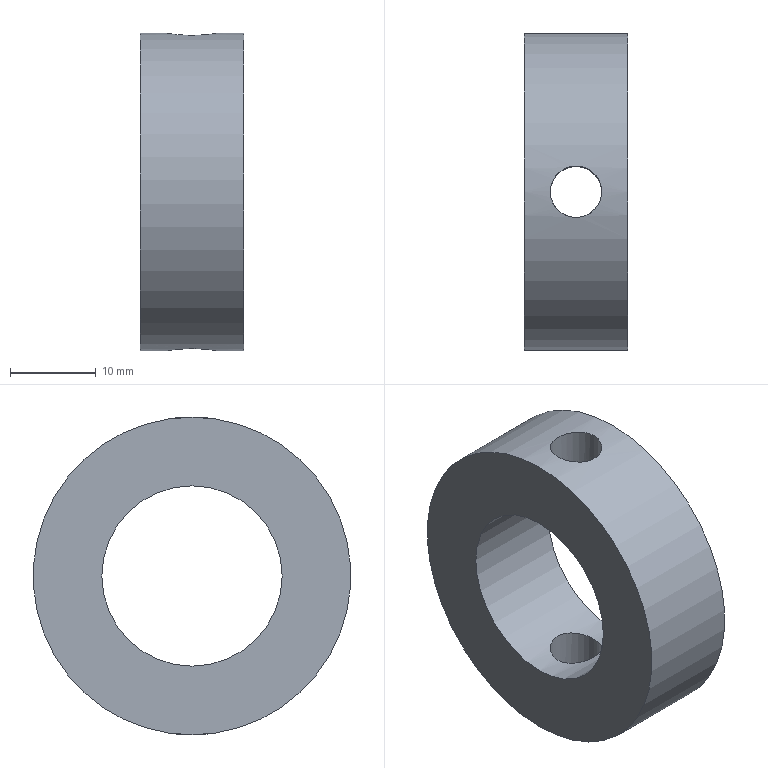Component | NX | RETAININGRING | 1 solid | 6 faces | volume 8291 mm3 | cylinder 4 | plane 2 | commonest cylinder face diameters 6 x2 37 x1 21 x1